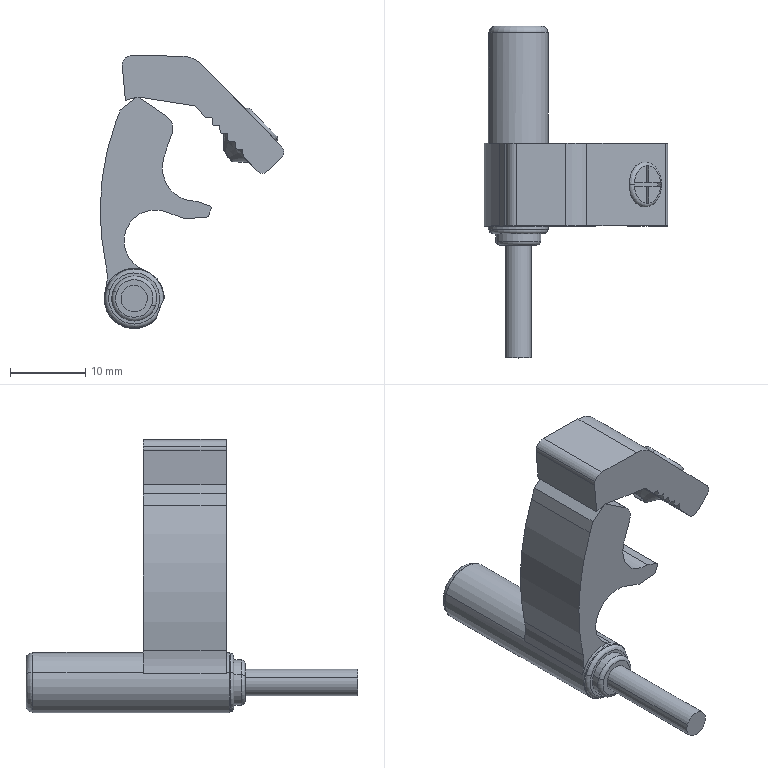Component | SolidWorks | AirTACCylinderFSC_80x75_S_FB-1_FCS1_A_SC80-1 | 1 solid | 100 faces | volume 4627 mm3 | plane 55 | cylinder 29 | torus 12 | cone 4 | commonest cylinder face diameters 6 x8 8 x3 8.9 x3 2.7 x2 3.5 x2 8.26 x2 0.6 x2 2 x2